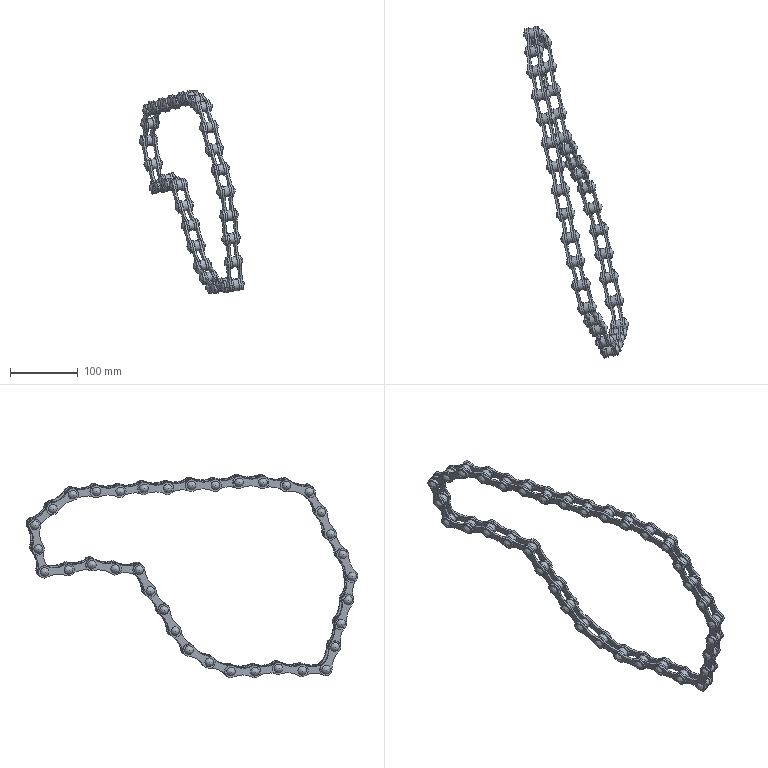Assembly | NX | mm | 180 component files | 180 solids | 1332 faces | box 155.28 x 489.73 x 300.09 mm | volume 229015 mm3 | cylinder 684 | plane 504 | spline 72 | cone 72 | commonest cylinder face diameters 7 x252 70.075 x144 18 x144 4 x72 15 x36 4.5 x36
Bill of materials:
unnamed part 1 | 36 |  | Plain cylindrical ring/sleeve: a solid of revolution with a smooth outer cylinder, two flat parallel end faces, and a single concentric cylindrical through bore.
unnamed part 2 | 36 |  | Solid stepped pin with a domed head: a dome-shaped head with a flat underside, a large-diameter cylindrical shank, a step down to a smaller-diameter section, and a short end section that tapers slightly with a small shoulder or ridge near the tip.
unnamed part 3 | 72 |  | Flat link plate of constant thickness with rounded (semicircular) ends, a waisted middle with concave side edges, and one round through hole near each end.
unnamed part 4 | 36 |  | Domed-head hollow shank: a dome-shaped head with a flat underside and a cylindrical tubular shank with a concentric bore that is open at the shank end.
Mates:
1. concentric | 2 1 | 1 1
2. concentric | 3 4 | 1_2 2
3. concentric | 3 3 | 1_2 2
4. concentric | 3 2 | 3 3
5. concentric | 3 1 | 3 4
6. concentric | 4 2 | 3 1
7. concentric | 1_2 1 | 3 4
8. concentric | 4 1 | 3 1
9. concentric | 4 1 | 3 2
10. concentric | 1_2__3_4 17 edge | 1_2__3_4 18 edge
11. concentric | 1_2__3_4 16 edge | 1_2__3_4 17 edge
12. concentric | 1_2__3_4 15 edge | 1_2__3_4 16 edge
13. concentric | 1_2__3_4 14 edge | 1_2__3_4 15 edge
14. concentric | 1_2__3_4 13 edge | 1_2__3_4 14 edge
15. concentric | 1_2__3_4 12 edge | 1_2__3_4 13 edge
16. concentric | 1_2__3_4 11 edge | 1_2__3_4 12 edge
17. concentric | 1_2__3_4 10 edge | 1_2__3_4 11 edge
18. concentric | 1_2__3_4 9 edge | 1_2__3_4 10 edge
19. concentric | 1_2__3_4 8 edge | 1_2__3_4 9 edge
20. concentric | 1_2__3_4 7 edge | 1_2__3_4 8 edge
21. concentric | 1_2__3_4 6 edge | 1_2__3_4 7 edge
22. concentric | 1_2__3_4 5 edge | 1_2__3_4 6 edge
23. concentric | 1_2__3_4 4 edge | 1_2__3_4 5 edge
24. concentric | 1_2__3_4 3 edge | 1_2__3_4 4 edge
25. concentric | 1_2__3_4 2 edge | 1_2__3_4 3 edge
26. concentric | 1_2__3_4 1 edge | 1_2__3_4 2 edge
27. concentric | 1_2__3_4 18 edge | 1_2__3_4 1 edge